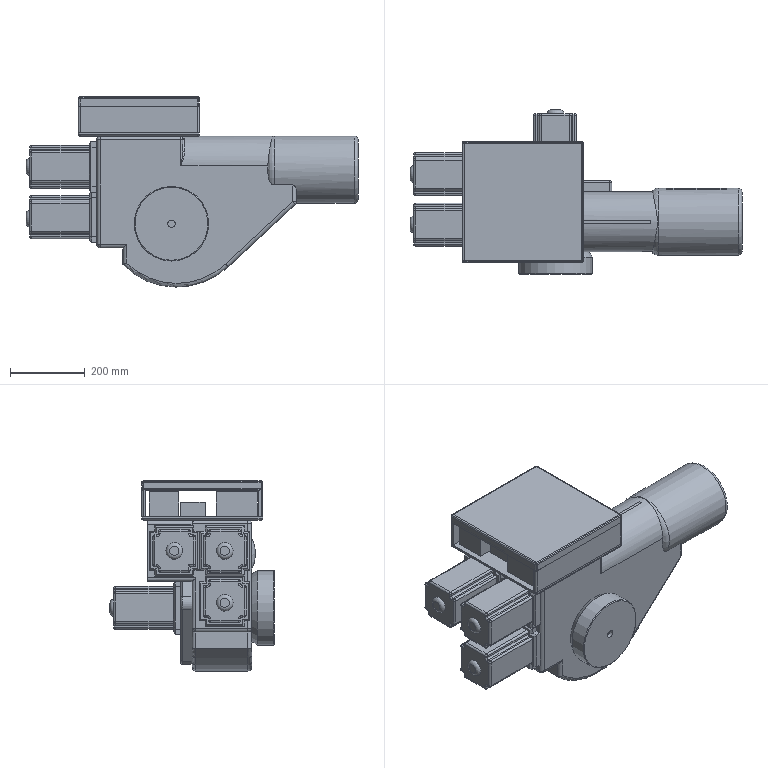Component | NX | 4_ELBOW_PIVOT | 18 solids | 600 faces | volume 52511592 mm3 | plane 320 | cylinder 195 | sphere 45 | torus 31 | spline 8 | cone 1 | commonest cylinder face diameters 10 x125 6 x36 20 x20 180 x5 50 x3 48.924 x1 405.565 x1 1000 x1